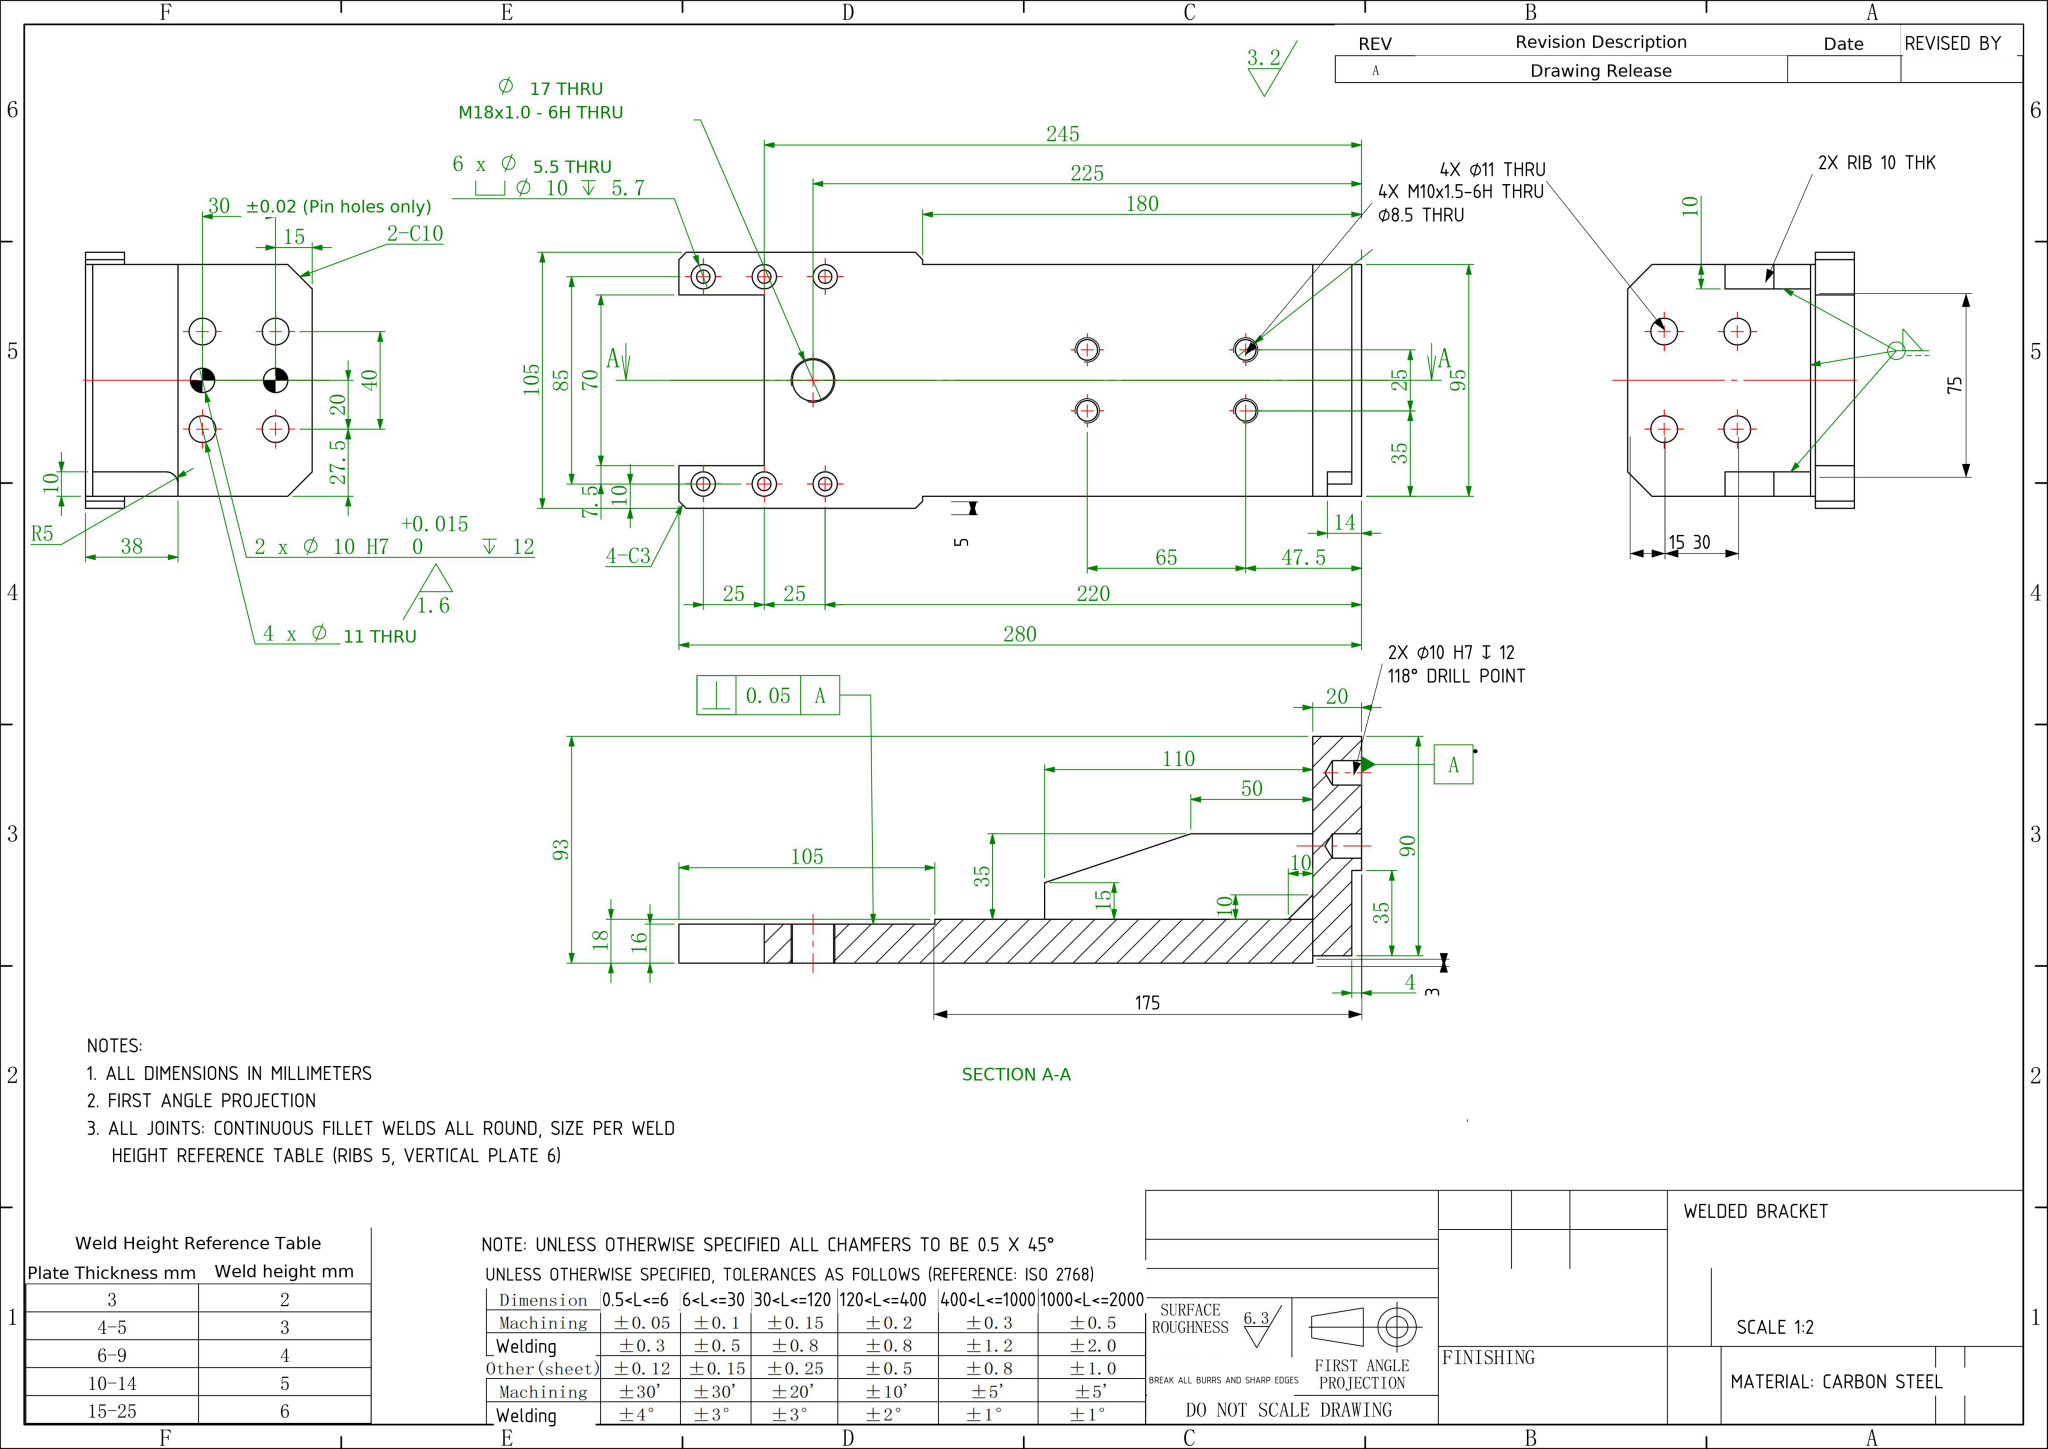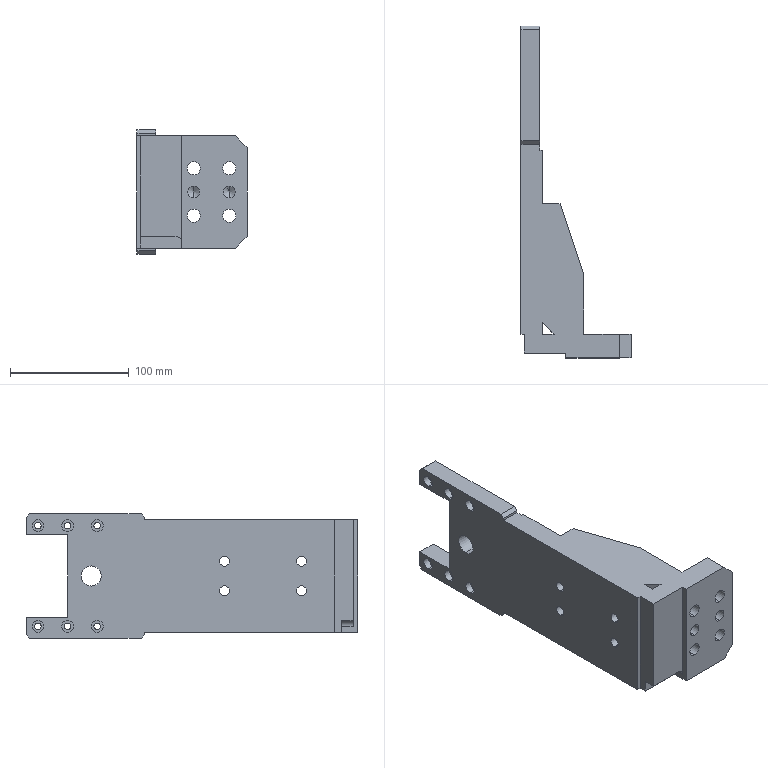Part | NX | mm | 1 solid | 97 faces | box 93 x 280 x 105 mm | volume 595899 mm3 | cylinder 47 | plane 46 | cone 4 | commonest cylinder face diameters 10 x17 5.5 x12 8.5 x8 11 x8 17 x2